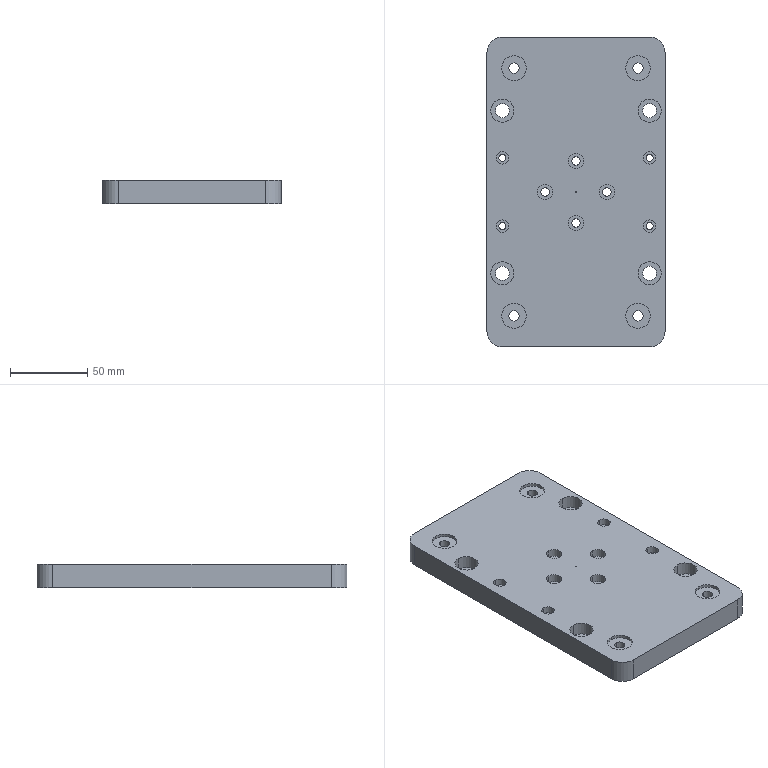Component | SolidWorks | DC-46-017-1 | 1 solid | 104 faces | box 115 x 200 x 15 mm | volume 326772 mm3 | cylinder 78 | plane 26 | commonest cylinder face diameters 16 x16 8 x8 4.5 x8 15 x8 10 x8 5.5 x8 9 x8 6.6 x8
build123d program:
from build123d import *

# Parameters (mm, degrees)
SKETCH1_W                                           = 200
SKETCH1_H                                           = 115
BOSS_EXTRUDE1_DEPTH                                 = 7.5
FILLET1_R                                           = 10
F_0_19_0_19_DIAMETER_HOLE1_D                        = 0.19
M5_HEX_SOCKET_HEAD_CAP_SCREW_CBORE1_D               = 5.5
M5_HEX_SOCKET_HEAD_CAP_SCREW_CBORE1_CBORE_D         = 10
M5_HEX_SOCKET_HEAD_CAP_SCREW_CBORE1_CBORE_DEPTH     = 5.4
M8_HEX_SOCKET_HEAD_CAP_SCREW_CBORE1_D               = 9
M8_HEX_SOCKET_HEAD_CAP_SCREW_CBORE1_CBORE_D         = 15
M8_HEX_SOCKET_HEAD_CAP_SCREW_CBORE1_CBORE_DEPTH     = 8.6
SKETCH9_R                                           = 8
CUT_EXTRUDE1_DEPTH                                  = 3
M6_CLEARANCE_HOLE1_D                                = 6.6
SKETCH12_R                                          = 8
CUT_EXTRUDE2_DEPTH                                  = 2
HOLE_SIZE_ACCORDING_TO_TYPE_1_OF_HEXAGO_D           = 4.5
HOLE_SIZE_ACCORDING_TO_TYPE_1_OF_HEXAGO_CBORE_D     = 8
HOLE_SIZE_ACCORDING_TO_TYPE_1_OF_HEXAGO_CBORE_DEPTH = 4.6


with BuildPart() as part:
    # Sketch1 → Boss-Extrude1 (new, symmetric)
    with BuildSketch(Plane.XY):
        Rectangle(SKETCH1_W, SKETCH1_H)
    extrude(amount=BOSS_EXTRUDE1_DEPTH, both=True)

    # Fillet1
    fillet1_edges = [part.edges().sort_by_distance(p)[0] for p in [
        (-100, 57.5, 0),
        (100, 57.5, 0),
        (100, -57.5, 0),
        (-100, -57.5, 0),
    ]]
    fillet(fillet1_edges, radius=FILLET1_R)

    # 0.19 _0.19_ Diameter Hole1 (through all)
    with Locations(Plane(origin=(0, 0, -7.5), x_dir=(-1, 0, 0), z_dir=(0, 0, -1))):
        with Locations((0, 0)):
            Hole(F_0_19_0_19_DIAMETER_HOLE1_D / 2)

    # M5 Hex Socket Head Cap Screw CBORE1 (through all)
    with Locations(Plane.XY.offset(7.5)):
        with Locations((20, 0), (0, 20), (-20, 0), (0, -20)):
            CounterBoreHole(M5_HEX_SOCKET_HEAD_CAP_SCREW_CBORE1_D / 2, M5_HEX_SOCKET_HEAD_CAP_SCREW_CBORE1_CBORE_D / 2, M5_HEX_SOCKET_HEAD_CAP_SCREW_CBORE1_CBORE_DEPTH)

    # M8 Hex Socket Head Cap Screw CBORE1 (through all)
    with Locations(Plane.XY.offset(7.5)):
        with Locations((52.5, -47.5), (-52.5, -47.5), (52.5, 47.5), (-52.5, 47.5)):
            CounterBoreHole(M8_HEX_SOCKET_HEAD_CAP_SCREW_CBORE1_D / 2, M8_HEX_SOCKET_HEAD_CAP_SCREW_CBORE1_CBORE_D / 2, M8_HEX_SOCKET_HEAD_CAP_SCREW_CBORE1_CBORE_DEPTH)

    # Sketch9 → Cut-Extrude1 (cut)
    with BuildSketch(Plane(origin=(0, 0, -7.5), x_dir=(-1, 0, 0), z_dir=(0, 0, -1))):
        with Locations((-52.5, 47.5)):
            Circle(SKETCH9_R)
        with Locations((52.5, 47.5)):
            Circle(SKETCH9_R)
        with Locations((-52.5, -47.5)):
            Circle(SKETCH9_R)
        with Locations((52.5, -47.5)):
            Circle(SKETCH9_R)
    extrude(amount=-CUT_EXTRUDE1_DEPTH, mode=Mode.SUBTRACT)

    # M6 Clearance Hole1 (through all)
    with Locations(Plane(origin=(0, 0, -7.5), x_dir=(-1, 0, 0), z_dir=(0, 0, -1))):
        with Locations((-80, 40), (80, 40), (80, -40), (-80, -40)):
            Hole(M6_CLEARANCE_HOLE1_D / 2)

    # Sketch12 → Cut-Extrude2 (cut)
    with BuildSketch(Plane.XY.offset(7.5)):
        with Locations((-80, 40)):
            Circle(SKETCH12_R)
        with Locations((-80, -40)):
            Circle(SKETCH12_R)
        with Locations((80, 40)):
            Circle(SKETCH12_R)
        with Locations((80, -40)):
            Circle(SKETCH12_R)
    extrude(amount=-CUT_EXTRUDE2_DEPTH, mode=Mode.SUBTRACT)

    # Hole Size_According to_ Type 1 of Hexago (through all)
    with Locations(Plane.XY.offset(7.5)):
        with Locations((22, 47.5), (-22, 47.5), (22, -47.5), (-22, -47.5)):
            CounterBoreHole(HOLE_SIZE_ACCORDING_TO_TYPE_1_OF_HEXAGO_D / 2, HOLE_SIZE_ACCORDING_TO_TYPE_1_OF_HEXAGO_CBORE_D / 2, HOLE_SIZE_ACCORDING_TO_TYPE_1_OF_HEXAGO_CBORE_DEPTH)


solid = part.part

# Placed as in the assembly
solid = solid.moved(Location((311.865, 195.227, 2083.133), (0, 0, 90)))